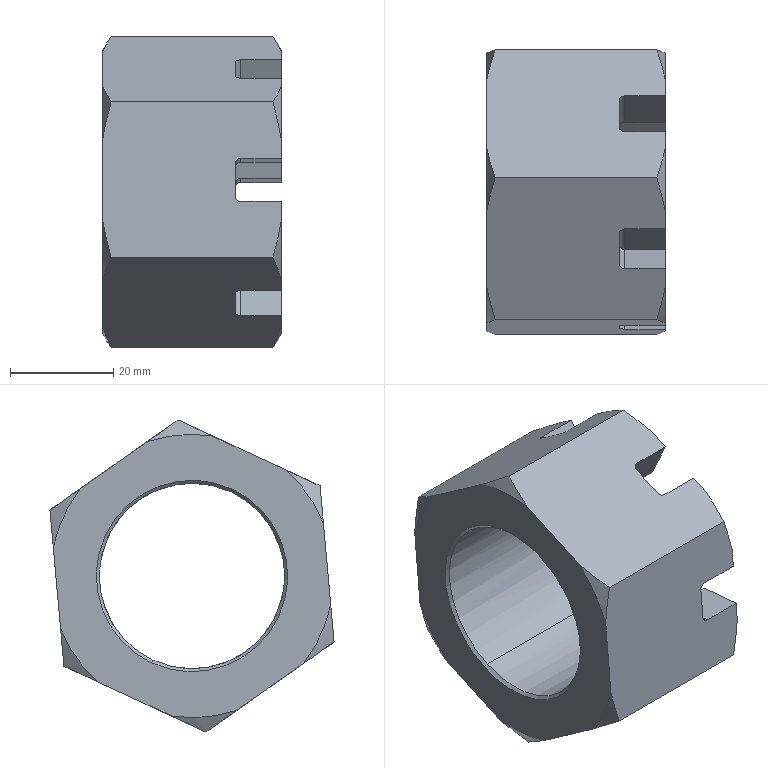Component | SolidWorks | GB_T9459-1988[HexSlottedThinNutFineThreadM36_3]-1 | 1 solid | 59 faces | volume 43974 mm3 | plane 31 | cone 14 | cylinder 14 | commonest cylinder face diameters 2.25 x12 36 x2